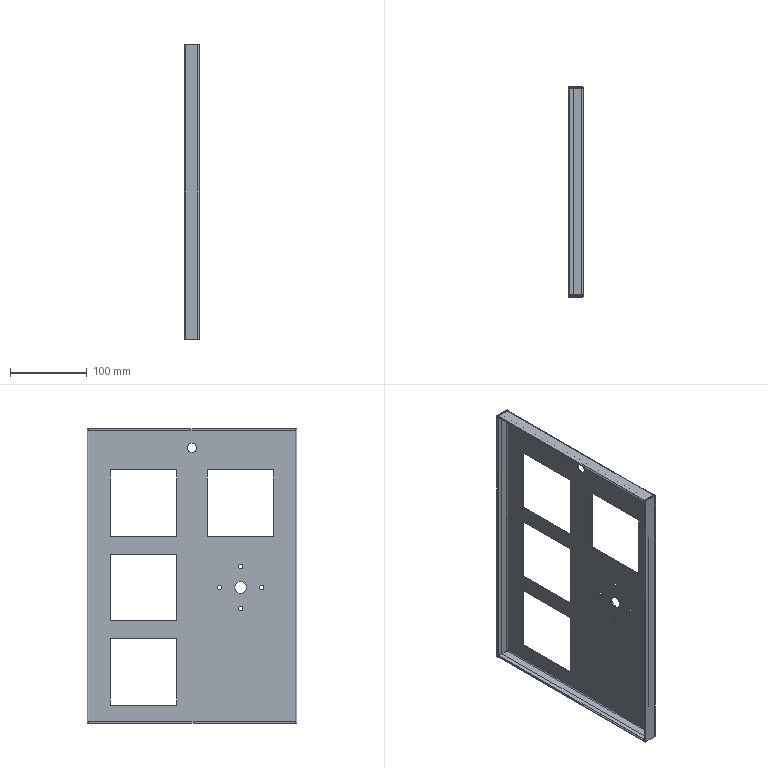Component | SolidWorks | MeteringChamberDoorAssembly-1_MeteringChamberDoorPanel-1 | 1 solid | 102 faces | volume 128371 mm3 | plane 74 | cylinder 28 | commonest cylinder face diameters 5.5 x8 4.8 x4 2.4 x4 2.5 x4 0.1 x4 12 x2 15 x2